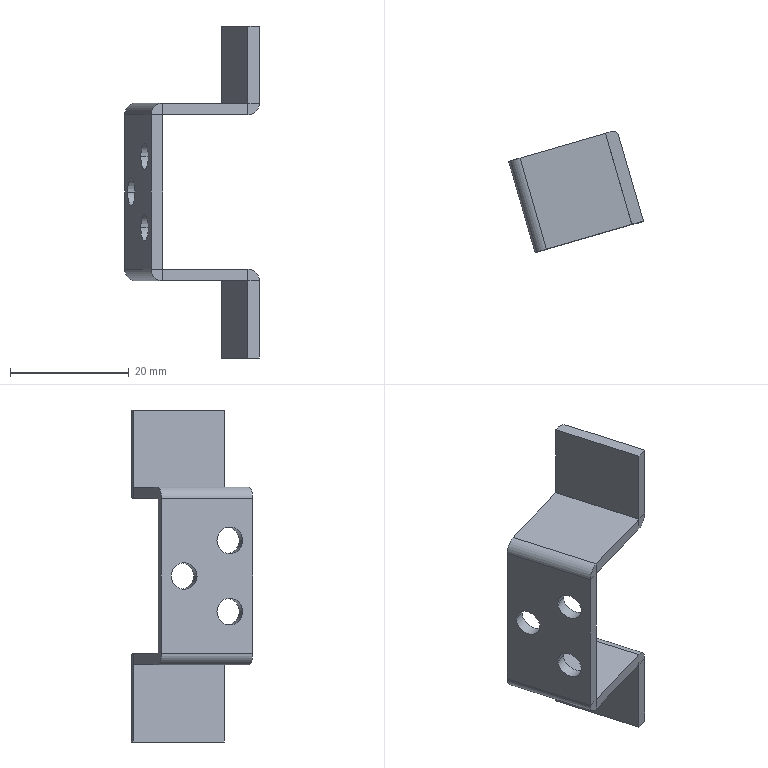Component | SolidWorks | LeftDoorAssembly-1_LockWeldBracket-1 | 1 solid | 46 faces | volume 2723 mm3 | plane 30 | cylinder 16 | commonest cylinder face diameters 4.5 x6 0.02 x4 4.02 x4 2 x2